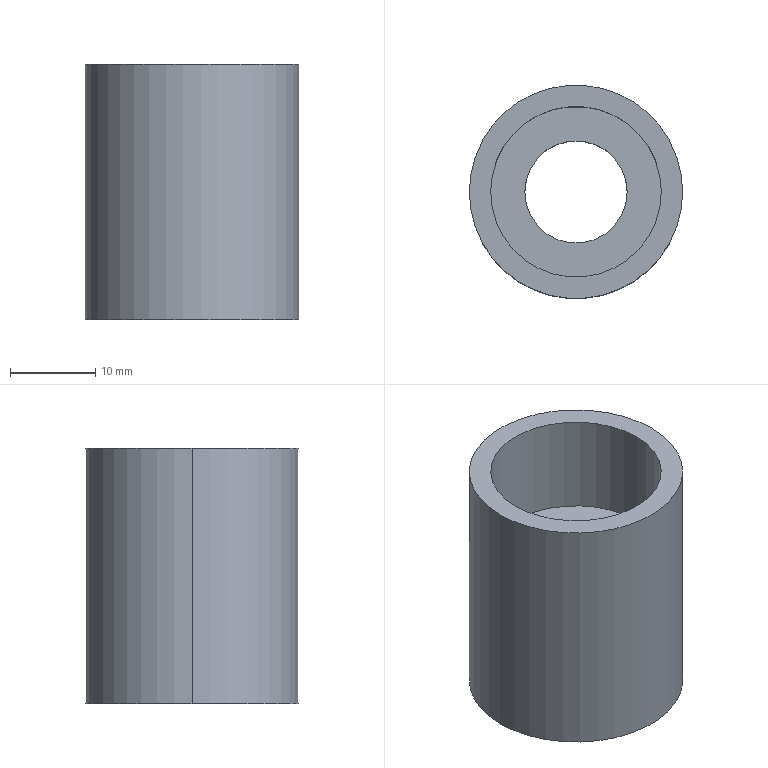Component | SolidWorks | DoubleFilmTransport-1_AdjustmentNut-1 | 1 solid | 9 faces | box 25 x 25 x 30 mm | volume 8921 mm3 | cylinder 6 | plane 3 | commonest cylinder face diameters 25 x2 12 x2 20 x2
build123d program:
from build123d import *


with BuildPart() as part:
    # Sketch1 → Revolve1 (revolve)
    with BuildSketch(Plane(origin=(0, 0, 0), x_dir=(-1, 0, 0), z_dir=(0, 0, -1)), mode=Mode.PRIVATE) as revolve1_sk:
        Polygon((-30, 10), (-18, 10), (-18, 6), (0, 6), (0, 12.5), (-30, 12.5), align=None)
    revolve(revolve1_sk.sketch.rotate(Axis((30, 0, 0), (-1, 0, 0)), 270), axis=Axis((30, 0, 0), (-1, 0, 0)))


solid = part.part

# Placed as in the assembly
solid = solid.moved(Location((-298.746, 95.373, 40.5), (0, -90, 0)))
STEP:
#1=CARTESIAN_POINT('',(-12.254,3.755,2.776));
#2=VERTEX_POINT('',#1);
#3=CARTESIAN_POINT('',(-11.27,3.755,2.776));
#4=VERTEX_POINT('',#3);
#5=CARTESIAN_POINT('',(-11.762,3.755,2.776));
#6=DIRECTION('',(0.,0.,-1.));
#7=DIRECTION('',(-1.,0.,0.));
#8=AXIS2_PLACEMENT_3D('',#5,#6,#7);
#9=CIRCLE('',#8,0.4921);
#10=EDGE_CURVE('',#2,#4,#9,.T.);
#11=ORIENTED_EDGE('',*,*,#10,.T.);
#12=CARTESIAN_POINT('',(-11.27,3.755,1.594));
#13=VERTEX_POINT('',#12);
#14=CARTESIAN_POINT('',(-11.27,3.755,2.776));
#15=DIRECTION('',(0.,0.,-1.));
#16=VECTOR('',#15,39.37);
#17=LINE('',#14,#16);
#18=EDGE_CURVE('',#4,#13,#17,.T.);
#19=ORIENTED_EDGE('',*,*,#18,.T.);
#20=CARTESIAN_POINT('',(-12.254,3.755,1.594));
#21=VERTEX_POINT('',#20);
#22=CARTESIAN_POINT('',(-11.762,3.755,1.594));
#23=DIRECTION('',(0.,0.,-1.));
#24=DIRECTION('',(-1.,0.,0.));
#25=AXIS2_PLACEMENT_3D('',#22,#23,#24);
#26=CIRCLE('',#25,0.4921);
#27=EDGE_CURVE('',#21,#13,#26,.T.);
#28=ORIENTED_EDGE('',*,*,#27,.F.);
#29=CARTESIAN_POINT('',(-12.254,3.755,2.776));
#30=DIRECTION('',(0.,0.,-1.));
#31=VECTOR('',#30,39.37);
#32=LINE('',#29,#31);
#33=EDGE_CURVE('',#2,#21,#32,.T.);
#34=ORIENTED_EDGE('',*,*,#33,.F.);
#35=EDGE_LOOP('',(#11,#19,#28,#34));
#36=FACE_OUTER_BOUND('',#35,.T.);
#37=CARTESIAN_POINT('',(-11.762,3.755,2.776));
#38=DIRECTION('',(0.,0.,-1.));
#39=DIRECTION('',(-1.,0.,0.));
#40=AXIS2_PLACEMENT_3D('',#37,#38,#39);
#41=CYLINDRICAL_SURFACE('',#40,0.4921);
#42=ADVANCED_FACE('',(#36),#41,.T.);
#43=CARTESIAN_POINT('',(-11.525,3.755,2.303));
#44=VERTEX_POINT('',#43);
#45=CARTESIAN_POINT('',(-11.998,3.755,2.303));
#46=VERTEX_POINT('',#45);
#47=CARTESIAN_POINT('',(-11.762,3.755,2.303));
#48=DIRECTION('',(0.,0.,-1.));
#49=DIRECTION('',(-1.,0.,0.));
#50=AXIS2_PLACEMENT_3D('',#47,#48,#49);
#51=CIRCLE('',#50,0.2362);
#52=EDGE_CURVE('',#44,#46,#51,.T.);
#53=ORIENTED_EDGE('',*,*,#52,.F.);
#54=CARTESIAN_POINT('',(-11.525,3.755,1.594));
#55=VERTEX_POINT('',#54);
#56=CARTESIAN_POINT('',(-11.525,3.755,2.776));
#57=DIRECTION('',(0.,0.,-1.));
#58=VECTOR('',#57,39.37);
#59=LINE('',#56,#58);
#60=EDGE_CURVE('',#44,#55,#59,.T.);
#61=ORIENTED_EDGE('',*,*,#60,.T.);
#62=CARTESIAN_POINT('',(-11.998,3.755,1.594));
#63=VERTEX_POINT('',#62);
#64=CARTESIAN_POINT('',(-11.762,3.755,1.594));
#65=DIRECTION('',(0.,0.,-1.));
#66=DIRECTION('',(-1.,0.,0.));
#67=AXIS2_PLACEMENT_3D('',#64,#65,#66);
#68=CIRCLE('',#67,0.2362);
#69=EDGE_CURVE('',#55,#63,#68,.T.);
#70=ORIENTED_EDGE('',*,*,#69,.T.);
#71=CARTESIAN_POINT('',(-11.998,3.755,2.776));
#72=DIRECTION('',(0.,0.,-1.));
#73=VECTOR('',#72,39.37);
#74=LINE('',#71,#73);
#75=EDGE_CURVE('',#46,#63,#74,.T.);
#76=ORIENTED_EDGE('',*,*,#75,.F.);
#77=EDGE_LOOP('',(#53,#61,#70,#76));
#78=FACE_OUTER_BOUND('',#77,.T.);
#79=CARTESIAN_POINT('',(-11.762,3.755,2.776));
#80=DIRECTION('',(0.,0.,-1.));
#81=DIRECTION('',(-1.,0.,0.));
#82=AXIS2_PLACEMENT_3D('',#79,#80,#81);
#83=CYLINDRICAL_SURFACE('',#82,0.2362);
#84=ADVANCED_FACE('',(#78),#83,.F.);
#85=CARTESIAN_POINT('',(-11.368,3.755,2.776));
#86=VERTEX_POINT('',#85);
#87=CARTESIAN_POINT('',(-12.155,3.755,2.776));
#88=VERTEX_POINT('',#87);
#89=CARTESIAN_POINT('',(-11.762,3.755,2.776));
#90=DIRECTION('',(0.,0.,-1.));
#91=DIRECTION('',(-1.,0.,0.));
#92=AXIS2_PLACEMENT_3D('',#89,#90,#91);
#93=CIRCLE('',#92,0.3937);
#94=EDGE_CURVE('',#86,#88,#93,.T.);
#95=ORIENTED_EDGE('',*,*,#94,.F.);
#96=CARTESIAN_POINT('',(-11.368,3.755,2.303));
#97=VERTEX_POINT('',#96);
#98=CARTESIAN_POINT('',(-11.368,3.755,2.776));
#99=DIRECTION('',(0.,0.,-1.));
#100=VECTOR('',#99,39.37);
#101=LINE('',#98,#100);
#102=EDGE_CURVE('',#86,#97,#101,.T.);
#103=ORIENTED_EDGE('',*,*,#102,.T.);
#104=CARTESIAN_POINT('',(-12.155,3.755,2.303));
#105=VERTEX_POINT('',#104);
#106=CARTESIAN_POINT('',(-11.762,3.755,2.303));
#107=DIRECTION('',(0.,0.,-1.));
#108=DIRECTION('',(-1.,0.,0.));
#109=AXIS2_PLACEMENT_3D('',#106,#107,#108);
#110=CIRCLE('',#109,0.3937);
#111=EDGE_CURVE('',#97,#105,#110,.T.);
#112=ORIENTED_EDGE('',*,*,#111,.T.);
#113=CARTESIAN_POINT('',(-12.155,3.755,2.776));
#114=DIRECTION('',(0.,0.,-1.));
#115=VECTOR('',#114,39.37);
#116=LINE('',#113,#115);
#117=EDGE_CURVE('',#88,#105,#116,.T.);
#118=ORIENTED_EDGE('',*,*,#117,.F.);
#119=EDGE_LOOP('',(#95,#103,#112,#118));
#120=FACE_OUTER_BOUND('',#119,.T.);
#121=CARTESIAN_POINT('',(-11.762,3.755,2.776));
#122=DIRECTION('',(0.,0.,-1.));
#123=DIRECTION('',(-1.,0.,0.));
#124=AXIS2_PLACEMENT_3D('',#121,#122,#123);
#125=CYLINDRICAL_SURFACE('',#124,0.3937);
#126=ADVANCED_FACE('',(#120),#125,.F.);
#127=CARTESIAN_POINT('',(-11.762,3.755,2.776));
#128=DIRECTION('',(0.,0.,-1.));
#129=DIRECTION('',(-1.,0.,0.));
#130=AXIS2_PLACEMENT_3D('',#127,#128,#129);
#131=CIRCLE('',#130,0.3937);
#132=EDGE_CURVE('',#88,#86,#131,.T.);
#133=ORIENTED_EDGE('',*,*,#132,.T.);
#134=ORIENTED_EDGE('',*,*,#94,.T.);
#135=EDGE_LOOP('',(#133,#134));
#136=FACE_BOUND('',#135,.T.);
#137=ORIENTED_EDGE('',*,*,#10,.F.);
#138=CARTESIAN_POINT('',(-11.762,3.755,2.776));
#139=DIRECTION('',(0.,0.,-1.));
#140=DIRECTION('',(-1.,0.,0.));
#141=AXIS2_PLACEMENT_3D('',#138,#139,#140);
#142=CIRCLE('',#141,0.4921);
#143=EDGE_CURVE('',#4,#2,#142,.T.);
#144=ORIENTED_EDGE('',*,*,#143,.F.);
#145=EDGE_LOOP('',(#137,#144));
#146=FACE_OUTER_BOUND('',#145,.T.);
#147=CARTESIAN_POINT('',(-11.762,4.247,2.776));
#148=DIRECTION('',(0.,0.,1.));
#149=DIRECTION('',(1.,0.,0.));
#150=AXIS2_PLACEMENT_3D('',#147,#148,#149);
#151=PLANE('',#150);
#152=ADVANCED_FACE('',(#136,#146),#151,.T.);
#153=ORIENTED_EDGE('',*,*,#102,.F.);
#154=ORIENTED_EDGE('',*,*,#132,.F.);
#155=ORIENTED_EDGE('',*,*,#117,.T.);
#156=CARTESIAN_POINT('',(-11.762,3.755,2.303));
#157=DIRECTION('',(0.,0.,-1.));
#158=DIRECTION('',(-1.,0.,0.));
#159=AXIS2_PLACEMENT_3D('',#156,#157,#158);
#160=CIRCLE('',#159,0.3937);
#161=EDGE_CURVE('',#105,#97,#160,.T.);
#162=ORIENTED_EDGE('',*,*,#161,.T.);
#163=EDGE_LOOP('',(#153,#154,#155,#162));
#164=FACE_OUTER_BOUND('',#163,.T.);
#165=CARTESIAN_POINT('',(-11.762,3.755,2.776));
#166=DIRECTION('',(0.,0.,-1.));
#167=DIRECTION('',(-1.,0.,0.));
#168=AXIS2_PLACEMENT_3D('',#165,#166,#167);
#169=CYLINDRICAL_SURFACE('',#168,0.3937);
#170=ADVANCED_FACE('',(#164),#169,.F.);
#171=CARTESIAN_POINT('',(-11.762,3.755,2.303));
#172=DIRECTION('',(0.,0.,-1.));
#173=DIRECTION('',(-1.,0.,0.));
#174=AXIS2_PLACEMENT_3D('',#171,#172,#173);
#175=CIRCLE('',#174,0.2362);
#176=EDGE_CURVE('',#46,#44,#175,.T.);
#177=ORIENTED_EDGE('',*,*,#176,.T.);
#178=ORIENTED_EDGE('',*,*,#52,.T.);
#179=EDGE_LOOP('',(#177,#178));
#180=FACE_BOUND('',#179,.T.);
#181=ORIENTED_EDGE('',*,*,#161,.F.);
#182=ORIENTED_EDGE('',*,*,#111,.F.);
#183=EDGE_LOOP('',(#181,#182));
#184=FACE_OUTER_BOUND('',#183,.T.);
#185=CARTESIAN_POINT('',(-11.762,4.149,2.303));
#186=DIRECTION('',(0.,0.,1.));
#187=DIRECTION('',(1.,0.,0.));
#188=AXIS2_PLACEMENT_3D('',#185,#186,#187);
#189=PLANE('',#188);
#190=ADVANCED_FACE('',(#180,#184),#189,.T.);
#191=ORIENTED_EDGE('',*,*,#60,.F.);
#192=ORIENTED_EDGE('',*,*,#176,.F.);
#193=ORIENTED_EDGE('',*,*,#75,.T.);
#194=CARTESIAN_POINT('',(-11.762,3.755,1.594));
#195=DIRECTION('',(0.,0.,-1.));
#196=DIRECTION('',(-1.,0.,0.));
#197=AXIS2_PLACEMENT_3D('',#194,#195,#196);
#198=CIRCLE('',#197,0.2362);
#199=EDGE_CURVE('',#63,#55,#198,.T.);
#200=ORIENTED_EDGE('',*,*,#199,.T.);
#201=EDGE_LOOP('',(#191,#192,#193,#200));
#202=FACE_OUTER_BOUND('',#201,.T.);
#203=CARTESIAN_POINT('',(-11.762,3.755,2.776));
#204=DIRECTION('',(0.,0.,-1.));
#205=DIRECTION('',(-1.,0.,0.));
#206=AXIS2_PLACEMENT_3D('',#203,#204,#205);
#207=CYLINDRICAL_SURFACE('',#206,0.2362);
#208=ADVANCED_FACE('',(#202),#207,.F.);
#209=ORIENTED_EDGE('',*,*,#27,.T.);
#210=CARTESIAN_POINT('',(-11.762,3.755,1.594));
#211=DIRECTION('',(0.,0.,-1.));
#212=DIRECTION('',(-1.,0.,0.));
#213=AXIS2_PLACEMENT_3D('',#210,#211,#212);
#214=CIRCLE('',#213,0.4921);
#215=EDGE_CURVE('',#13,#21,#214,.T.);
#216=ORIENTED_EDGE('',*,*,#215,.T.);
#217=EDGE_LOOP('',(#209,#216));
#218=FACE_OUTER_BOUND('',#217,.T.);
#219=ORIENTED_EDGE('',*,*,#199,.F.);
#220=ORIENTED_EDGE('',*,*,#69,.F.);
#221=EDGE_LOOP('',(#219,#220));
#222=FACE_BOUND('',#221,.T.);
#223=CARTESIAN_POINT('',(-11.762,3.991,1.594));
#224=DIRECTION('',(0.,0.,-1.));
#225=DIRECTION('',(-1.,0.,0.));
#226=AXIS2_PLACEMENT_3D('',#223,#224,#225);
#227=PLANE('',#226);
#228=ADVANCED_FACE('',(#218,#222),#227,.T.);
#229=ORIENTED_EDGE('',*,*,#18,.F.);
#230=ORIENTED_EDGE('',*,*,#143,.T.);
#231=ORIENTED_EDGE('',*,*,#33,.T.);
#232=ORIENTED_EDGE('',*,*,#215,.F.);
#233=EDGE_LOOP('',(#229,#230,#231,#232));
#234=FACE_OUTER_BOUND('',#233,.T.);
#235=CARTESIAN_POINT('',(-11.762,3.755,2.776));
#236=DIRECTION('',(0.,0.,-1.));
#237=DIRECTION('',(-1.,0.,0.));
#238=AXIS2_PLACEMENT_3D('',#235,#236,#237);
#239=CYLINDRICAL_SURFACE('',#238,0.4921);
#240=ADVANCED_FACE('',(#234),#239,.T.);
#241=CLOSED_SHELL('',(#42,#84,#126,#152,#170,#190,#208,#228,#240));
#242=MANIFOLD_SOLID_BREP('',#241);
#243=CARTESIAN_POINT('',(0.,0.,0.));
#244=DIRECTION('',(0.,0.,1.));
#245=DIRECTION('',(1.,0.,0.));
#246=AXIS2_PLACEMENT_3D('',#243,#244,#245);
#247=(LENGTH_UNIT()NAMED_UNIT(*)SI_UNIT($,.METRE.));
#248=LENGTH_MEASURE_WITH_UNIT(LENGTH_MEASURE(0.0254),#247);
#249=DIMENSIONAL_EXPONENTS(1.,0.,0.,0.,0.,0.,0.);
#250=(CONVERSION_BASED_UNIT('',#248)LENGTH_UNIT()NAMED_UNIT(#249));
#251=UNCERTAINTY_MEASURE_WITH_UNIT(LENGTH_MEASURE(0.00001),#250,'','');
#252=(NAMED_UNIT(*)PLANE_ANGLE_UNIT()SI_UNIT($,.RADIAN.));
#253=(NAMED_UNIT(*)SI_UNIT($,.STERADIAN.)SOLID_ANGLE_UNIT());
#254=(GEOMETRIC_REPRESENTATION_CONTEXT(3)GLOBAL_UNCERTAINTY_ASSIGNED_CONTEXT((#251))GLOBAL_UNIT_ASSIGNED_CONTEXT((#250,#252,#253))REPRESENTATION_CONTEXT('',''));
#255=ADVANCED_BREP_SHAPE_REPRESENTATION('',(#242,#246),#254);
#256=COLOUR_RGB('',0.7922,0.8196,0.9333);
#257=FILL_AREA_STYLE_COLOUR('',#256);
#258=FILL_AREA_STYLE('',(#257));
#259=SURFACE_STYLE_FILL_AREA(#258);
#260=SURFACE_SIDE_STYLE('',(#259));
#261=SURFACE_STYLE_USAGE(.BOTH.,#260);
#262=PRESENTATION_STYLE_ASSIGNMENT((#261));
#263=STYLED_ITEM('',(#262),#242);
#264=(LENGTH_UNIT()NAMED_UNIT(*)SI_UNIT($,.METRE.));
#265=LENGTH_MEASURE_WITH_UNIT(LENGTH_MEASURE(0.0254),#264);
#266=DIMENSIONAL_EXPONENTS(1.,0.,0.,0.,0.,0.,0.);
#267=(CONVERSION_BASED_UNIT('',#265)LENGTH_UNIT()NAMED_UNIT(#266));
#268=UNCERTAINTY_MEASURE_WITH_UNIT(LENGTH_MEASURE(0.00001),#267,'','');
#269=(NAMED_UNIT(*)PLANE_ANGLE_UNIT()SI_UNIT($,.RADIAN.));
#270=(NAMED_UNIT(*)SI_UNIT($,.STERADIAN.)SOLID_ANGLE_UNIT());
#271=(GEOMETRIC_REPRESENTATION_CONTEXT(3)GLOBAL_UNCERTAINTY_ASSIGNED_CONTEXT((#268))GLOBAL_UNIT_ASSIGNED_CONTEXT((#267,#269,#270))REPRESENTATION_CONTEXT('',''));
#272=MECHANICAL_DESIGN_GEOMETRIC_PRESENTATION_REPRESENTATION('',(#263),#271);
#273=PRESENTATION_LAYER_ASSIGNMENT('','',(#263));